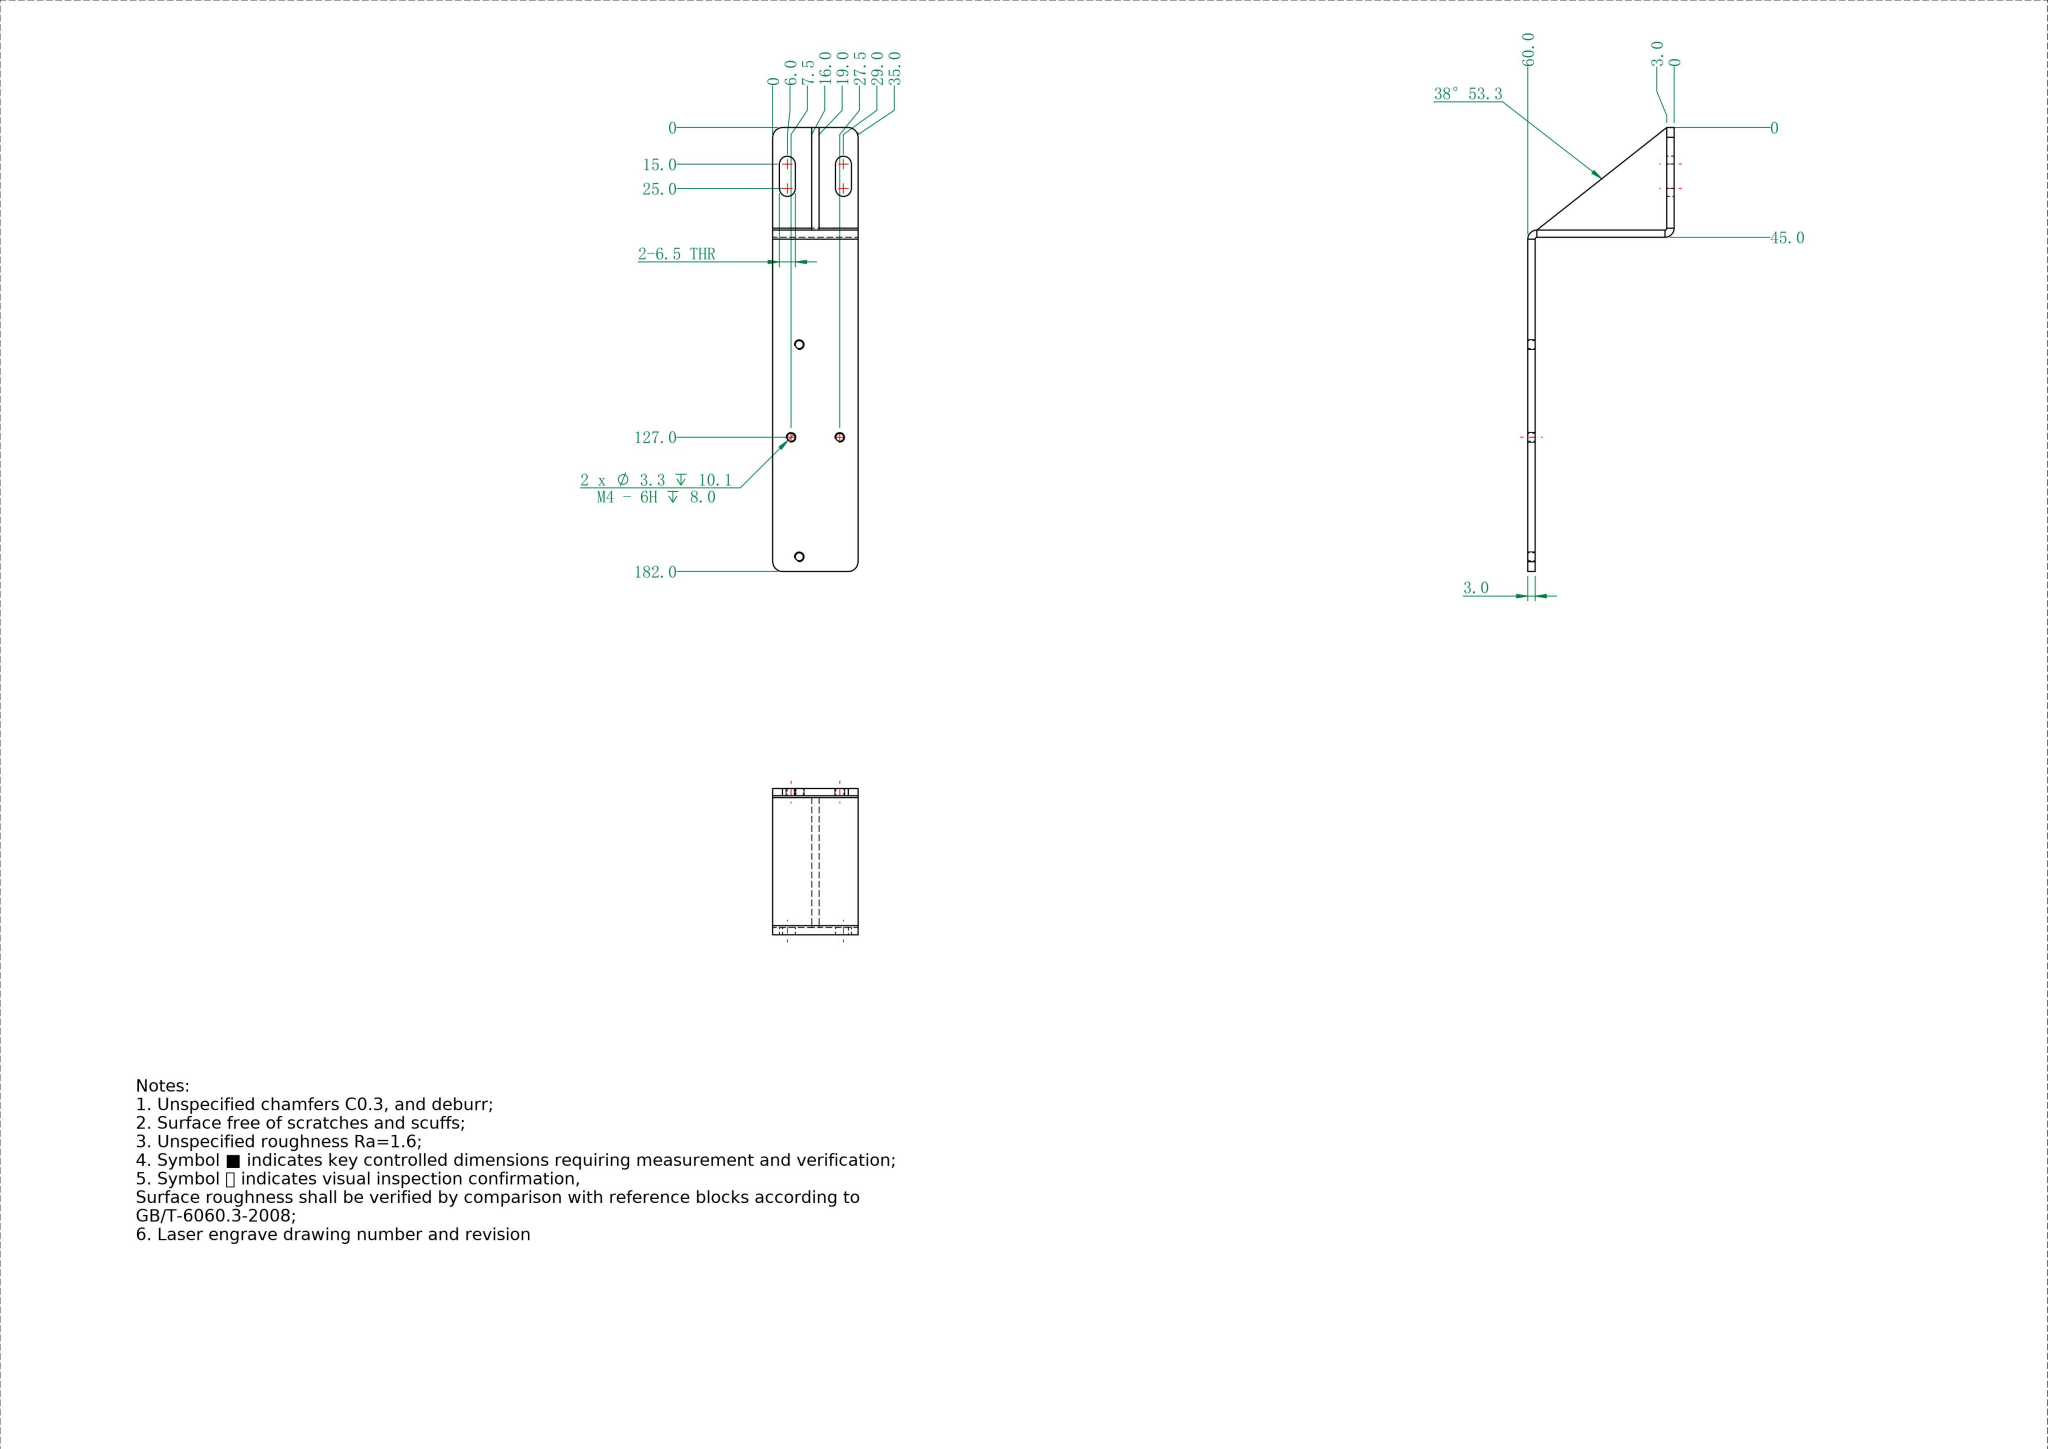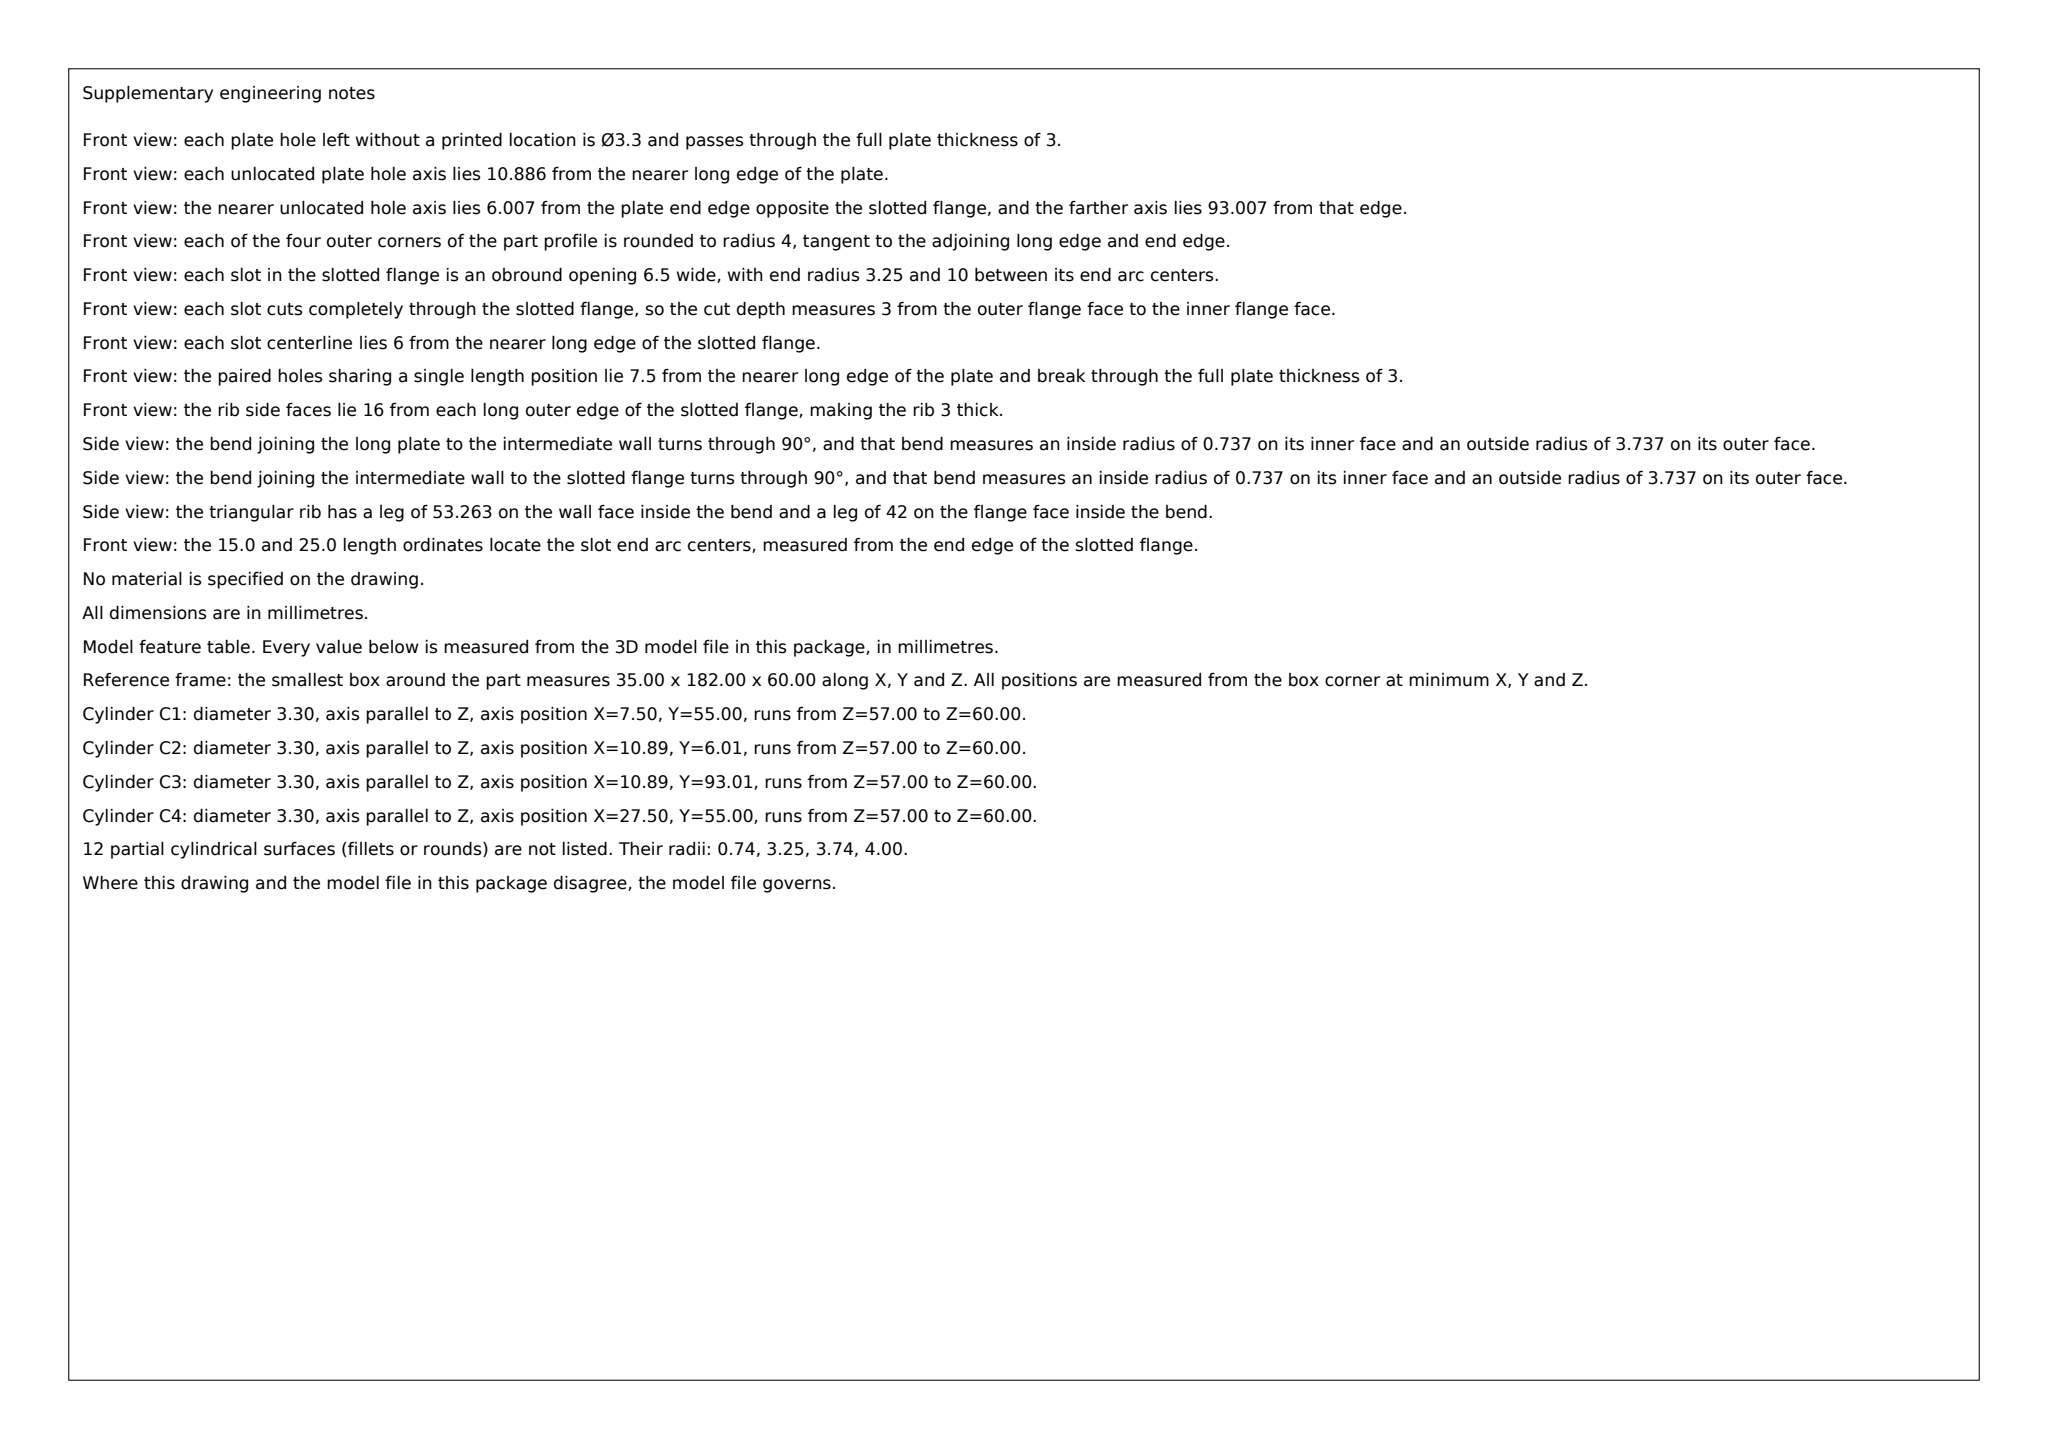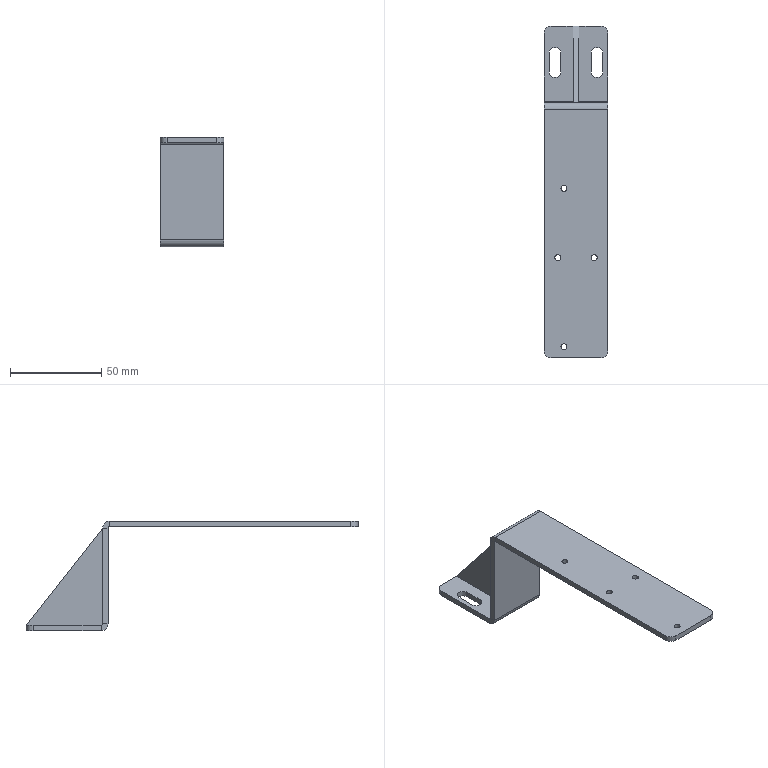Part | SolidWorks | mm | 1 solid | 48 faces | box 35 x 182 x 60 mm | volume 27516 mm3 | plane 27 | cylinder 21 | commonest cylinder face diameters 3.3 x8 8 x4 6.5 x4 1.473 x3 7.473 x2
Drawing notes:
2X Ø3.3 THRU, 10.9 FROM EDGE, 89.0 & 176.0 FROM TOP | from the solid: cyl dia 3.3 axis z at (10.89,93.01) and (10.89,6.01), len 3.0 = full 3 mm wall; 182-93.01=89.0, 182-6.01=176.0
2X R0.7 BEND RAD (BOTH 90 DEG BENDS) | from the solid: Two 90 deg bends: planes y=137/140 and z=57/60 with 3.0 thk; no other fillets listed (fillet_radii empty), bend rad per drawing R0.7